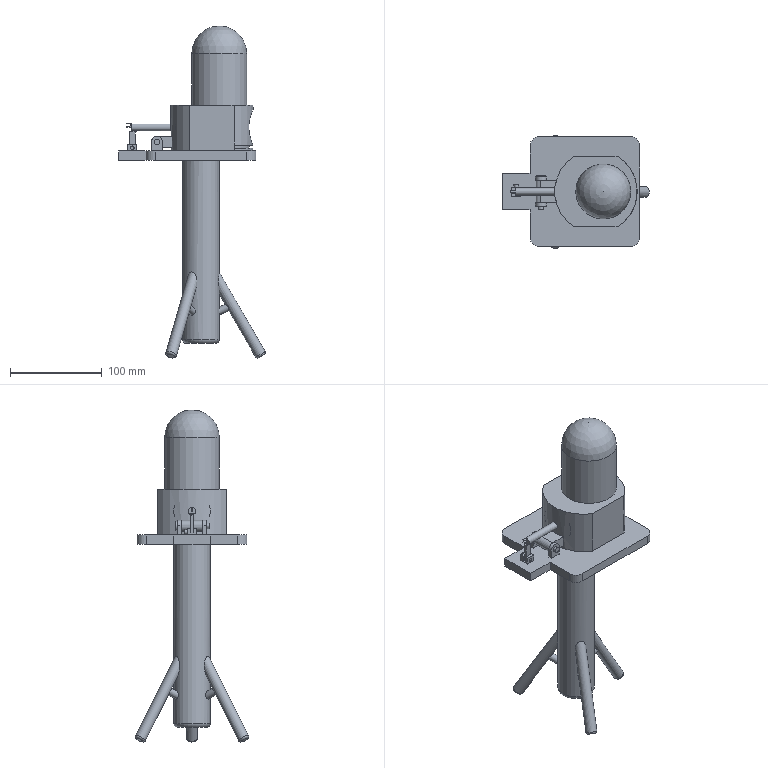Assembly | NX | mm | 8 component files | 8 solids | 137 faces | box 160.46 x 123.79 x 362.56 mm | volume 784038 mm3 | plane 90 | cylinder 40 | torus 4 | sphere 2 | cone 1 | commonest cylinder face diameters 4 x6 12 x6 8 x6 6 x4 20 x4 40 x3 90 x3 36 x2
Bill of materials:
unnamed part 1 | 1 |  | Solid stepped cylinder: a long plain shank with a shorter, larger-diameter cylindrical head at one end.
unnamed part 2 | 1 |  | Thin flat circular disc with a central round bore that has a single small rectangular keyway notch.
unnamed part 3 | 1 |  | Headed cylindrical pin: a long slender round shank with a thin, larger-diameter flat disc head at one end.
unnamed part 4 | 1 |  | Rectangular bar or link with a round through-hole near one end and a small angled, lip-like projection along the top edge at the other end.
unnamed part 5 | 1 |  | Long solid round shaft with an axial keyway slot near one end and a reduced, notched flat tang at the other end.
unnamed part 6 | 1 |  | Compact, roughly cylindrical housing block with one flattened side. It has a large vertical bore with an annular recess on top, a large horizontal cross-bore through the side, a small eyelet tab with a hole, and a small central hole on the bottom face.
unnamed part 7 | 1 |  | Solid cylinder with a hemispherical (domed) end and a flat opposite end, i.e. a bullet or capsule-end shape.
unnamed part 8 | 1 |  | Stand-like structure: a square top plate with rounded corners and a rectangular side extension, a central vertical cylindrical column below it, and three splayed round rod legs joined to the column by short struts. Small holed lugs stand on the top plate.
Mates:
1. fix | sheji-waiguan-2 1 component
2. touch align | sheji_-2 1 face | sheji-waiguan-2 1 face
3. touch align | sheji-waiguan-1 1 face | sheji_-2 1 face
4. touch align | she_ji-5 1 face | sheji-waiguan-2 1 face
5. touch align | she_ji-5 1 face | sheji-waiguan-2 1 face
6. touch align | sheji-waiguan-2 1 face | sheji_-2 1 face
7. touch align | she_ji-6 1 face | sheji_-2 1 face
8. touch align | sheji-waiguan-1 1 face | sheji_-2 1 face
9. touch align | she_ji-7 1 face | sheji_-2 1 face
10. touch align | she_ji-7 1 face | she_ji-6 1 face
11. touch align | she_ji-6 1 face | she_ji-7 1 face
12. parallel | sheji_-2 1 face | sheji-waiguan-2 1 face
13. touch align | sheji-waiguan-3 1 face | sheji-waiguan-2 1 face
14. touch align | sheji-waiguan-2 1 face | sheji-waiguan-3 1 face
15. touch align | sheji-waiguan-3 1 face | sheji-waiguan-2 1 face
16. touch align | sheji-waiguan-4 1 face | sheji-waiguan-2 1 face
17. touch align | sheji-waiguan-4 1 face | sheji-waiguan-2 1 face